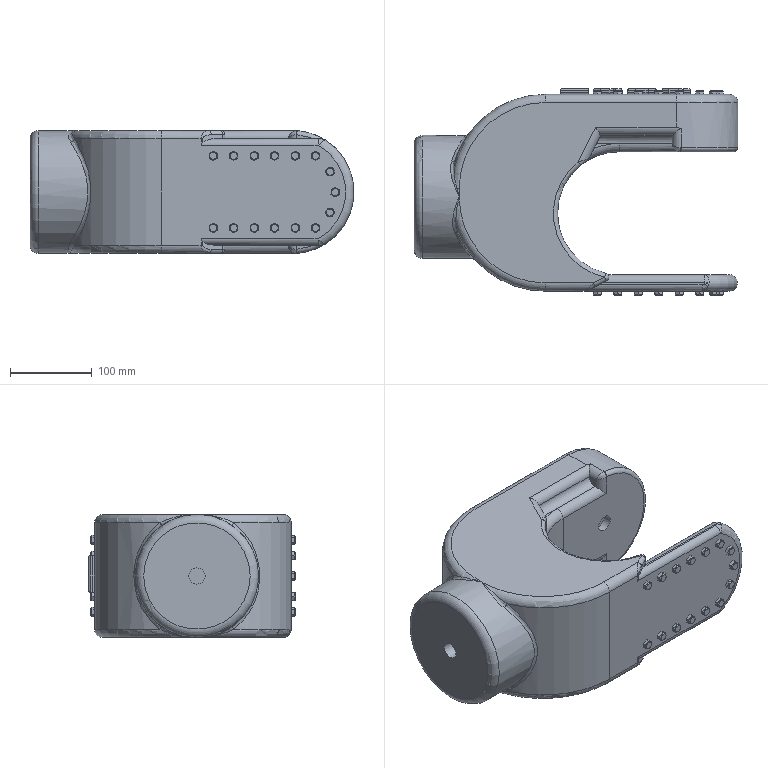Component | NX | 5_FOREARM | 35 solids | 516 faces | volume 7666754 mm3 | plane 314 | cylinder 132 | cone 30 | spline 22 | torus 12 | sphere 6 | commonest cylinder face diameters 4 x89 20 x27 10 x5 1 x4 150 x3 230 x2 16 x2